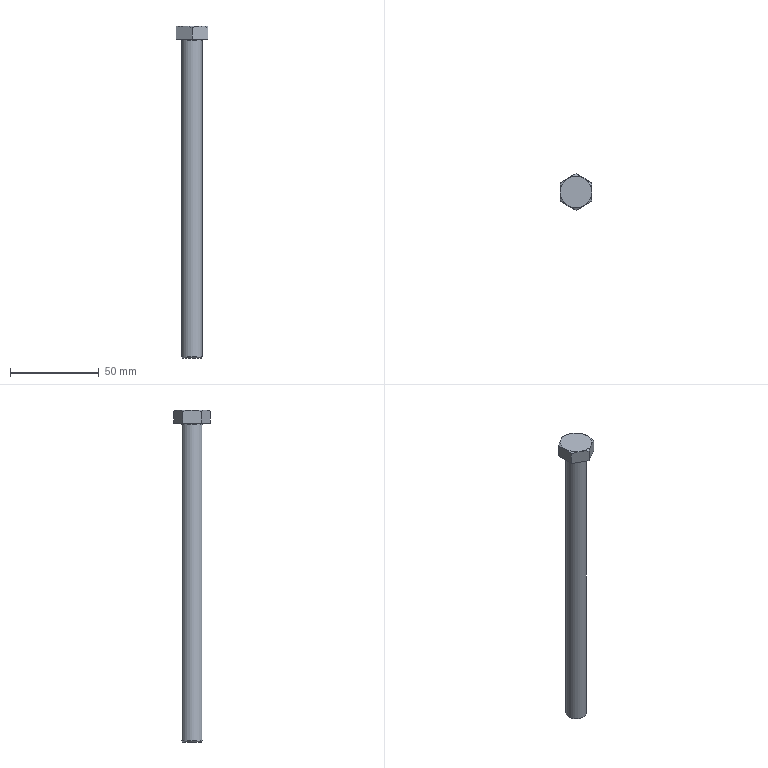Component | NX | BOLT_M12X170 | 1 solid | 18 faces | volume 21451 mm3 | plane 9 | cone 7 | cylinder 1 | torus 1 | commonest cylinder face diameters 11.701 x1